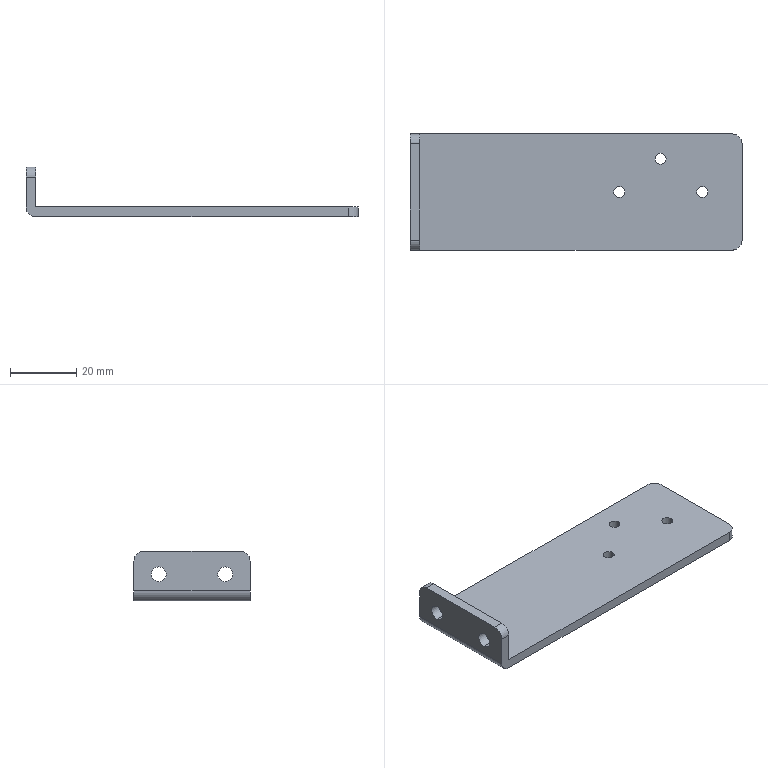Component | SolidWorks | H2020022-0443-1-1 | 1 solid | 23 faces | box 100 x 35 x 15 mm | volume 11497 mm3 | cylinder 15 | plane 8 | commonest cylinder face diameters 3.3 x6 6 x5 4.5 x4 | material Stainless Steel304
build123d program:
from build123d import *

# Parameters (mm, degrees)
BOSS_EXTRUDE1_DEPTH = 35
FILLET1_R           = 3
SKETCH2_R           = 2.25
CUT_EXTRUDE1_DEPTH  = 105.207
M4_TAPPED_HOLE1_D   = 3.3


with BuildPart() as part:
    # Sketch1 → Boss-Extrude1 (new body)
    with BuildSketch(Plane(origin=(0, 0, 0), x_dir=(1, 0, 0), z_dir=(0, 1, 0))):
        Polygon((0, 0), (0, -100), (-3, -100), (-3, -3), (-15, -3), (-15, 0), align=None)
    extrude(amount=BOSS_EXTRUDE1_DEPTH)

    # Fillet1
    fillet1_edges = [part.edges().sort_by_distance(p)[0] for p in [
        (0, 17.5, 0),
        (-1.5, 35, 100),
        (-1.5, 0, 100),
        (-15, 35, 1.5),
        (-15, 0, 1.5),
    ]]
    fillet(fillet1_edges, radius=FILLET1_R)

    # Sketch2 → Cut-Extrude1 (cut, through all)
    with BuildSketch(Plane.XY.offset(3)):
        with Locations((-8, 27.5)):
            Circle(SKETCH2_R)
        with Locations((-8, 7.5)):
            Circle(SKETCH2_R)
    extrude(amount=-CUT_EXTRUDE1_DEPTH, mode=Mode.SUBTRACT)

    # M4 Tapped Hole1 (through all)
    with Locations(Plane.ZY.offset(3)):
        with Locations((88, 17.5), (63, 17.5), (75.5, 27.5)):
            Hole(M4_TAPPED_HOLE1_D / 2)


solid = part.part

# Placed as in the assembly
solid = solid.moved(Location((11.932, 58.313, 375.197), (0, 90, 0)))
STEP:
#1=COLOUR_RGB('',0.7922,0.8196,0.9333);
#2=FILL_AREA_STYLE_COLOUR('',#1);
#3=FILL_AREA_STYLE('',(#2));
#4=SURFACE_STYLE_FILL_AREA(#3);
#5=SURFACE_SIDE_STYLE('',(#4));
#6=SURFACE_STYLE_USAGE(.BOTH.,#5);
#7=PRESENTATION_STYLE_ASSIGNMENT((#6));
#8=CARTESIAN_POINT('',(3.869,2.985,14.772));
#9=VERTEX_POINT('',#8);
#10=CARTESIAN_POINT('',(3.999,2.985,14.772));
#11=VERTEX_POINT('',#10);
#12=CARTESIAN_POINT('',(3.934,2.985,14.772));
#13=DIRECTION('',(-0.,0.,1.));
#14=DIRECTION('',(1.,0.,0.));
#15=AXIS2_PLACEMENT_3D('',#12,#13,#14);
#16=CIRCLE('',#15,0.06496);
#17=EDGE_CURVE('',#9,#11,#16,.T.);
#18=ORIENTED_EDGE('',*,*,#17,.F.);
#19=CARTESIAN_POINT('',(3.869,2.985,14.89));
#20=VERTEX_POINT('',#19);
#21=CARTESIAN_POINT('',(3.869,2.985,14.89));
#22=DIRECTION('',(-0.,0.,1.));
#23=VECTOR('',#22,39.37);
#24=LINE('',#21,#23);
#25=EDGE_CURVE('',#9,#20,#24,.T.);
#26=ORIENTED_EDGE('',*,*,#25,.T.);
#27=CARTESIAN_POINT('',(3.999,2.985,14.89));
#28=VERTEX_POINT('',#27);
#29=CARTESIAN_POINT('',(3.934,2.985,14.89));
#30=DIRECTION('',(-0.,0.,1.));
#31=DIRECTION('',(1.,0.,0.));
#32=AXIS2_PLACEMENT_3D('',#29,#30,#31);
#33=CIRCLE('',#32,0.06496);
#34=EDGE_CURVE('',#20,#28,#33,.T.);
#35=ORIENTED_EDGE('',*,*,#34,.T.);
#36=CARTESIAN_POINT('',(3.999,2.985,14.89));
#37=DIRECTION('',(-0.,0.,1.));
#38=VECTOR('',#37,39.37);
#39=LINE('',#36,#38);
#40=EDGE_CURVE('',#11,#28,#39,.T.);
#41=ORIENTED_EDGE('',*,*,#40,.F.);
#42=EDGE_LOOP('',(#18,#26,#35,#41));
#43=FACE_OUTER_BOUND('',#42,.T.);
#44=CARTESIAN_POINT('',(3.934,2.985,14.89));
#45=DIRECTION('',(-0.,0.,1.));
#46=DIRECTION('',(1.,0.,0.));
#47=AXIS2_PLACEMENT_3D('',#44,#45,#46);
#48=CYLINDRICAL_SURFACE('',#47,0.06496);
#49=ADVANCED_FACE('',(#43),#48,.F.);
#50=CARTESIAN_POINT('',(2.885,2.985,14.772));
#51=VERTEX_POINT('',#50);
#52=CARTESIAN_POINT('',(3.015,2.985,14.772));
#53=VERTEX_POINT('',#52);
#54=CARTESIAN_POINT('',(2.95,2.985,14.772));
#55=DIRECTION('',(-0.,0.,1.));
#56=DIRECTION('',(1.,0.,0.));
#57=AXIS2_PLACEMENT_3D('',#54,#55,#56);
#58=CIRCLE('',#57,0.06496);
#59=EDGE_CURVE('',#51,#53,#58,.T.);
#60=ORIENTED_EDGE('',*,*,#59,.F.);
#61=CARTESIAN_POINT('',(2.885,2.985,14.89));
#62=VERTEX_POINT('',#61);
#63=CARTESIAN_POINT('',(2.885,2.985,14.89));
#64=DIRECTION('',(-0.,0.,1.));
#65=VECTOR('',#64,39.37);
#66=LINE('',#63,#65);
#67=EDGE_CURVE('',#51,#62,#66,.T.);
#68=ORIENTED_EDGE('',*,*,#67,.T.);
#69=CARTESIAN_POINT('',(3.015,2.985,14.89));
#70=VERTEX_POINT('',#69);
#71=CARTESIAN_POINT('',(2.95,2.985,14.89));
#72=DIRECTION('',(-0.,0.,1.));
#73=DIRECTION('',(1.,0.,0.));
#74=AXIS2_PLACEMENT_3D('',#71,#72,#73);
#75=CIRCLE('',#74,0.06496);
#76=EDGE_CURVE('',#62,#70,#75,.T.);
#77=ORIENTED_EDGE('',*,*,#76,.T.);
#78=CARTESIAN_POINT('',(3.015,2.985,14.89));
#79=DIRECTION('',(-0.,0.,1.));
#80=VECTOR('',#79,39.37);
#81=LINE('',#78,#80);
#82=EDGE_CURVE('',#53,#70,#81,.T.);
#83=ORIENTED_EDGE('',*,*,#82,.F.);
#84=EDGE_LOOP('',(#60,#68,#77,#83));
#85=FACE_OUTER_BOUND('',#84,.T.);
#86=CARTESIAN_POINT('',(2.95,2.985,14.89));
#87=DIRECTION('',(-0.,0.,1.));
#88=DIRECTION('',(1.,0.,0.));
#89=AXIS2_PLACEMENT_3D('',#86,#87,#88);
#90=CYLINDRICAL_SURFACE('',#89,0.06496);
#91=ADVANCED_FACE('',(#85),#90,.F.);
#92=CARTESIAN_POINT('',(3.377,3.378,14.772));
#93=VERTEX_POINT('',#92);
#94=CARTESIAN_POINT('',(3.507,3.378,14.772));
#95=VERTEX_POINT('',#94);
#96=CARTESIAN_POINT('',(3.442,3.378,14.772));
#97=DIRECTION('',(-0.,0.,1.));
#98=DIRECTION('',(1.,0.,0.));
#99=AXIS2_PLACEMENT_3D('',#96,#97,#98);
#100=CIRCLE('',#99,0.06496);
#101=EDGE_CURVE('',#93,#95,#100,.T.);
#102=ORIENTED_EDGE('',*,*,#101,.F.);
#103=CARTESIAN_POINT('',(3.377,3.378,14.89));
#104=VERTEX_POINT('',#103);
#105=CARTESIAN_POINT('',(3.377,3.378,14.89));
#106=DIRECTION('',(-0.,0.,1.));
#107=VECTOR('',#106,39.37);
#108=LINE('',#105,#107);
#109=EDGE_CURVE('',#93,#104,#108,.T.);
#110=ORIENTED_EDGE('',*,*,#109,.T.);
#111=CARTESIAN_POINT('',(3.507,3.378,14.89));
#112=VERTEX_POINT('',#111);
#113=CARTESIAN_POINT('',(3.442,3.378,14.89));
#114=DIRECTION('',(-0.,0.,1.));
#115=DIRECTION('',(1.,0.,0.));
#116=AXIS2_PLACEMENT_3D('',#113,#114,#115);
#117=CIRCLE('',#116,0.06496);
#118=EDGE_CURVE('',#104,#112,#117,.T.);
#119=ORIENTED_EDGE('',*,*,#118,.T.);
#120=CARTESIAN_POINT('',(3.507,3.378,14.89));
#121=DIRECTION('',(-0.,0.,1.));
#122=VECTOR('',#121,39.37);
#123=LINE('',#120,#122);
#124=EDGE_CURVE('',#95,#112,#123,.T.);
#125=ORIENTED_EDGE('',*,*,#124,.F.);
#126=EDGE_LOOP('',(#102,#110,#119,#125));
#127=FACE_OUTER_BOUND('',#126,.T.);
#128=CARTESIAN_POINT('',(3.442,3.378,14.89));
#129=DIRECTION('',(-0.,0.,1.));
#130=DIRECTION('',(1.,0.,0.));
#131=AXIS2_PLACEMENT_3D('',#128,#129,#130);
#132=CYLINDRICAL_SURFACE('',#131,0.06496);
#133=ADVANCED_FACE('',(#127),#132,.F.);
#134=CARTESIAN_POINT('',(0.4697,3.378,15.175));
#135=VERTEX_POINT('',#134);
#136=CARTESIAN_POINT('',(0.4697,3.378,14.998));
#137=VERTEX_POINT('',#136);
#138=CARTESIAN_POINT('',(0.4697,3.378,15.086));
#139=DIRECTION('',(1.,0.,0.));
#140=DIRECTION('',(0.,0.,-1.));
#141=AXIS2_PLACEMENT_3D('',#138,#139,#140);
#142=CIRCLE('',#141,0.08858);
#143=EDGE_CURVE('',#135,#137,#142,.T.);
#144=ORIENTED_EDGE('',*,*,#143,.F.);
#145=CARTESIAN_POINT('',(0.5879,3.378,15.175));
#146=VERTEX_POINT('',#145);
#147=CARTESIAN_POINT('',(0.4697,3.378,15.175));
#148=DIRECTION('',(1.,0.,0.));
#149=VECTOR('',#148,39.37);
#150=LINE('',#147,#149);
#151=EDGE_CURVE('',#135,#146,#150,.T.);
#152=ORIENTED_EDGE('',*,*,#151,.T.);
#153=CARTESIAN_POINT('',(0.5879,3.378,14.998));
#154=VERTEX_POINT('',#153);
#155=CARTESIAN_POINT('',(0.5879,3.378,15.086));
#156=DIRECTION('',(1.,0.,0.));
#157=DIRECTION('',(0.,0.,-1.));
#158=AXIS2_PLACEMENT_3D('',#155,#156,#157);
#159=CIRCLE('',#158,0.08858);
#160=EDGE_CURVE('',#146,#154,#159,.T.);
#161=ORIENTED_EDGE('',*,*,#160,.T.);
#162=CARTESIAN_POINT('',(0.4697,3.378,14.998));
#163=DIRECTION('',(1.,0.,0.));
#164=VECTOR('',#163,39.37);
#165=LINE('',#162,#164);
#166=EDGE_CURVE('',#137,#154,#165,.T.);
#167=ORIENTED_EDGE('',*,*,#166,.F.);
#168=EDGE_LOOP('',(#144,#152,#161,#167));
#169=FACE_OUTER_BOUND('',#168,.T.);
#170=CARTESIAN_POINT('',(0.4697,3.378,15.086));
#171=DIRECTION('',(1.,0.,0.));
#172=DIRECTION('',(0.,0.,-1.));
#173=AXIS2_PLACEMENT_3D('',#170,#171,#172);
#174=CYLINDRICAL_SURFACE('',#173,0.08858);
#175=ADVANCED_FACE('',(#169),#174,.F.);
#176=CARTESIAN_POINT('',(0.4697,2.591,15.175));
#177=VERTEX_POINT('',#176);
#178=CARTESIAN_POINT('',(0.4697,2.591,14.998));
#179=VERTEX_POINT('',#178);
#180=CARTESIAN_POINT('',(0.4697,2.591,15.086));
#181=DIRECTION('',(1.,0.,0.));
#182=DIRECTION('',(0.,0.,-1.));
#183=AXIS2_PLACEMENT_3D('',#180,#181,#182);
#184=CIRCLE('',#183,0.08858);
#185=EDGE_CURVE('',#177,#179,#184,.T.);
#186=ORIENTED_EDGE('',*,*,#185,.F.);
#187=CARTESIAN_POINT('',(0.5879,2.591,15.175));
#188=VERTEX_POINT('',#187);
#189=CARTESIAN_POINT('',(0.4697,2.591,15.175));
#190=DIRECTION('',(1.,0.,0.));
#191=VECTOR('',#190,39.37);
#192=LINE('',#189,#191);
#193=EDGE_CURVE('',#177,#188,#192,.T.);
#194=ORIENTED_EDGE('',*,*,#193,.T.);
#195=CARTESIAN_POINT('',(0.5879,2.591,14.998));
#196=VERTEX_POINT('',#195);
#197=CARTESIAN_POINT('',(0.5879,2.591,15.086));
#198=DIRECTION('',(1.,0.,0.));
#199=DIRECTION('',(0.,0.,-1.));
#200=AXIS2_PLACEMENT_3D('',#197,#198,#199);
#201=CIRCLE('',#200,0.08858);
#202=EDGE_CURVE('',#188,#196,#201,.T.);
#203=ORIENTED_EDGE('',*,*,#202,.T.);
#204=CARTESIAN_POINT('',(0.4697,2.591,14.998));
#205=DIRECTION('',(1.,0.,0.));
#206=VECTOR('',#205,39.37);
#207=LINE('',#204,#206);
#208=EDGE_CURVE('',#179,#196,#207,.T.);
#209=ORIENTED_EDGE('',*,*,#208,.F.);
#210=EDGE_LOOP('',(#186,#194,#203,#209));
#211=FACE_OUTER_BOUND('',#210,.T.);
#212=CARTESIAN_POINT('',(0.4697,2.591,15.086));
#213=DIRECTION('',(1.,0.,0.));
#214=DIRECTION('',(0.,0.,-1.));
#215=AXIS2_PLACEMENT_3D('',#212,#213,#214);
#216=CYLINDRICAL_SURFACE('',#215,0.08858);
#217=ADVANCED_FACE('',(#211),#216,.F.);
#218=CARTESIAN_POINT('',(0.4697,3.378,15.086));
#219=DIRECTION('',(1.,0.,0.));
#220=DIRECTION('',(0.,0.,-1.));
#221=AXIS2_PLACEMENT_3D('',#218,#219,#220);
#222=CIRCLE('',#221,0.08858);
#223=EDGE_CURVE('',#137,#135,#222,.T.);
#224=ORIENTED_EDGE('',*,*,#223,.T.);
#225=ORIENTED_EDGE('',*,*,#143,.T.);
#226=EDGE_LOOP('',(#224,#225));
#227=FACE_BOUND('',#226,.T.);
#228=CARTESIAN_POINT('',(0.4697,2.591,15.086));
#229=DIRECTION('',(1.,0.,0.));
#230=DIRECTION('',(0.,0.,-1.));
#231=AXIS2_PLACEMENT_3D('',#228,#229,#230);
#232=CIRCLE('',#231,0.08858);
#233=EDGE_CURVE('',#179,#177,#232,.T.);
#234=ORIENTED_EDGE('',*,*,#233,.T.);
#235=ORIENTED_EDGE('',*,*,#185,.T.);
#236=EDGE_LOOP('',(#234,#235));
#237=FACE_BOUND('',#236,.T.);
#238=CARTESIAN_POINT('',(0.4697,2.296,14.89));
#239=VERTEX_POINT('',#238);
#240=CARTESIAN_POINT('',(0.4697,2.296,15.244));
#241=VERTEX_POINT('',#240);
#242=CARTESIAN_POINT('',(0.4697,2.296,15.362));
#243=DIRECTION('',(-0.,0.,1.));
#244=VECTOR('',#243,39.37);
#245=LINE('',#242,#244);
#246=EDGE_CURVE('',#239,#241,#245,.T.);
#247=ORIENTED_EDGE('',*,*,#246,.T.);
#248=CARTESIAN_POINT('',(0.4697,2.414,15.362));
#249=VERTEX_POINT('',#248);
#250=CARTESIAN_POINT('',(0.4697,2.414,15.244));
#251=DIRECTION('',(-1.,-0.,-0.));
#252=DIRECTION('',(0.,0.,-1.));
#253=AXIS2_PLACEMENT_3D('',#250,#251,#252);
#254=CIRCLE('',#253,0.1181);
#255=EDGE_CURVE('',#241,#249,#254,.T.);
#256=ORIENTED_EDGE('',*,*,#255,.T.);
#257=CARTESIAN_POINT('',(0.4697,3.556,15.362));
#258=VERTEX_POINT('',#257);
#259=CARTESIAN_POINT('',(0.4697,3.674,15.362));
#260=DIRECTION('',(0.,-1.,0.));
#261=VECTOR('',#260,39.37);
#262=LINE('',#259,#261);
#263=EDGE_CURVE('',#258,#249,#262,.T.);
#264=ORIENTED_EDGE('',*,*,#263,.F.);
#265=CARTESIAN_POINT('',(0.4697,3.674,15.244));
#266=VERTEX_POINT('',#265);
#267=CARTESIAN_POINT('',(0.4697,3.556,15.244));
#268=DIRECTION('',(-1.,-0.,-0.));
#269=DIRECTION('',(0.,0.,-1.));
#270=AXIS2_PLACEMENT_3D('',#267,#268,#269);
#271=CIRCLE('',#270,0.1181);
#272=EDGE_CURVE('',#258,#266,#271,.T.);
#273=ORIENTED_EDGE('',*,*,#272,.T.);
#274=CARTESIAN_POINT('',(0.4697,3.674,14.89));
#275=VERTEX_POINT('',#274);
#276=CARTESIAN_POINT('',(0.4697,3.674,15.362));
#277=DIRECTION('',(-0.,0.,1.));
#278=VECTOR('',#277,39.37);
#279=LINE('',#276,#278);
#280=EDGE_CURVE('',#275,#266,#279,.T.);
#281=ORIENTED_EDGE('',*,*,#280,.F.);
#282=CARTESIAN_POINT('',(0.4697,3.674,14.89));
#283=DIRECTION('',(0.,-1.,0.));
#284=VECTOR('',#283,39.37);
#285=LINE('',#282,#284);
#286=EDGE_CURVE('',#275,#239,#285,.T.);
#287=ORIENTED_EDGE('',*,*,#286,.T.);
#288=EDGE_LOOP('',(#247,#256,#264,#273,#281,#287));
#289=FACE_OUTER_BOUND('',#288,.T.);
#290=CARTESIAN_POINT('',(0.4697,3.674,15.362));
#291=DIRECTION('',(1.,0.,0.));
#292=DIRECTION('',(0.,-0.,-1.));
#293=AXIS2_PLACEMENT_3D('',#290,#291,#292);
#294=PLANE('',#293);
#295=ADVANCED_FACE('',(#227,#237,#289),#294,.F.);
#296=ORIENTED_EDGE('',*,*,#263,.T.);
#297=CARTESIAN_POINT('',(0.5879,2.414,15.362));
#298=VERTEX_POINT('',#297);
#299=CARTESIAN_POINT('',(0.5879,2.414,15.362));
#300=DIRECTION('',(1.,0.,0.));
#301=VECTOR('',#300,39.37);
#302=LINE('',#299,#301);
#303=EDGE_CURVE('',#249,#298,#302,.T.);
#304=ORIENTED_EDGE('',*,*,#303,.T.);
#305=CARTESIAN_POINT('',(0.5879,3.556,15.362));
#306=VERTEX_POINT('',#305);
#307=CARTESIAN_POINT('',(0.5879,3.674,15.362));
#308=DIRECTION('',(0.,-1.,0.));
#309=VECTOR('',#308,39.37);
#310=LINE('',#307,#309);
#311=EDGE_CURVE('',#306,#298,#310,.T.);
#312=ORIENTED_EDGE('',*,*,#311,.F.);
#313=CARTESIAN_POINT('',(0.5879,3.556,15.362));
#314=DIRECTION('',(-1.,-0.,-0.));
#315=VECTOR('',#314,39.37);
#316=LINE('',#313,#315);
#317=EDGE_CURVE('',#306,#258,#316,.T.);
#318=ORIENTED_EDGE('',*,*,#317,.T.);
#319=EDGE_LOOP('',(#296,#304,#312,#318));
#320=FACE_OUTER_BOUND('',#319,.T.);
#321=CARTESIAN_POINT('',(0.5879,3.674,15.362));
#322=DIRECTION('',(0.,-0.,-1.));
#323=DIRECTION('',(-1.,-0.,-0.));
#324=AXIS2_PLACEMENT_3D('',#321,#322,#323);
#325=PLANE('',#324);
#326=ADVANCED_FACE('',(#320),#325,.F.);
#327=CARTESIAN_POINT('',(0.5879,3.378,15.086));
#328=DIRECTION('',(1.,0.,0.));
#329=DIRECTION('',(0.,0.,-1.));
#330=AXIS2_PLACEMENT_3D('',#327,#328,#329);
#331=CIRCLE('',#330,0.08858);
#332=EDGE_CURVE('',#154,#146,#331,.T.);
#333=ORIENTED_EDGE('',*,*,#332,.F.);
#334=ORIENTED_EDGE('',*,*,#160,.F.);
#335=EDGE_LOOP('',(#333,#334));
#336=FACE_BOUND('',#335,.T.);
#337=CARTESIAN_POINT('',(0.5879,2.591,15.086));
#338=DIRECTION('',(1.,0.,0.));
#339=DIRECTION('',(0.,0.,-1.));
#340=AXIS2_PLACEMENT_3D('',#337,#338,#339);
#341=CIRCLE('',#340,0.08858);
#342=EDGE_CURVE('',#196,#188,#341,.T.);
#343=ORIENTED_EDGE('',*,*,#342,.F.);
#344=ORIENTED_EDGE('',*,*,#202,.F.);
#345=EDGE_LOOP('',(#343,#344));
#346=FACE_BOUND('',#345,.T.);
#347=ORIENTED_EDGE('',*,*,#311,.T.);
#348=CARTESIAN_POINT('',(0.5879,2.296,15.244));
#349=VERTEX_POINT('',#348);
#350=CARTESIAN_POINT('',(0.5879,2.414,15.244));
#351=DIRECTION('',(1.,0.,-0.));
#352=DIRECTION('',(0.,0.,1.));
#353=AXIS2_PLACEMENT_3D('',#350,#351,#352);
#354=CIRCLE('',#353,0.1181);
#355=EDGE_CURVE('',#298,#349,#354,.T.);
#356=ORIENTED_EDGE('',*,*,#355,.T.);
#357=CARTESIAN_POINT('',(0.5879,2.296,14.89));
#358=VERTEX_POINT('',#357);
#359=CARTESIAN_POINT('',(0.5879,2.296,14.89));
#360=DIRECTION('',(-0.,-0.,-1.));
#361=VECTOR('',#360,39.37);
#362=LINE('',#359,#361);
#363=EDGE_CURVE('',#349,#358,#362,.T.);
#364=ORIENTED_EDGE('',*,*,#363,.T.);
#365=CARTESIAN_POINT('',(0.5879,3.674,14.89));
#366=VERTEX_POINT('',#365);
#367=CARTESIAN_POINT('',(0.5879,3.674,14.89));
#368=DIRECTION('',(0.,-1.,0.));
#369=VECTOR('',#368,39.37);
#370=LINE('',#367,#369);
#371=EDGE_CURVE('',#366,#358,#370,.T.);
#372=ORIENTED_EDGE('',*,*,#371,.F.);
#373=CARTESIAN_POINT('',(0.5879,3.674,15.244));
#374=VERTEX_POINT('',#373);
#375=CARTESIAN_POINT('',(0.5879,3.674,14.89));
#376=DIRECTION('',(-0.,-0.,-1.));
#377=VECTOR('',#376,39.37);
#378=LINE('',#375,#377);
#379=EDGE_CURVE('',#374,#366,#378,.T.);
#380=ORIENTED_EDGE('',*,*,#379,.F.);
#381=CARTESIAN_POINT('',(0.5879,3.556,15.244));
#382=DIRECTION('',(1.,0.,-0.));
#383=DIRECTION('',(0.,0.,1.));
#384=AXIS2_PLACEMENT_3D('',#381,#382,#383);
#385=CIRCLE('',#384,0.1181);
#386=EDGE_CURVE('',#374,#306,#385,.T.);
#387=ORIENTED_EDGE('',*,*,#386,.T.);
#388=EDGE_LOOP('',(#347,#356,#364,#372,#380,#387));
#389=FACE_OUTER_BOUND('',#388,.T.);
#390=CARTESIAN_POINT('',(0.5879,3.674,14.89));
#391=DIRECTION('',(-1.,-0.,0.));
#392=DIRECTION('',(0.,0.,1.));
#393=AXIS2_PLACEMENT_3D('',#390,#391,#392);
#394=PLANE('',#393);
#395=ADVANCED_FACE('',(#336,#346,#389),#394,.F.);
#396=CARTESIAN_POINT('',(3.934,2.985,14.89));
#397=DIRECTION('',(-0.,0.,1.));
#398=DIRECTION('',(1.,0.,0.));
#399=AXIS2_PLACEMENT_3D('',#396,#397,#398);
#400=CIRCLE('',#399,0.06496);
#401=EDGE_CURVE('',#28,#20,#400,.T.);
#402=ORIENTED_EDGE('',*,*,#401,.F.);
#403=ORIENTED_EDGE('',*,*,#34,.F.);
#404=EDGE_LOOP('',(#402,#403));
#405=FACE_BOUND('',#404,.T.);
#406=CARTESIAN_POINT('',(2.95,2.985,14.89));
#407=DIRECTION('',(-0.,0.,1.));
#408=DIRECTION('',(1.,0.,0.));
#409=AXIS2_PLACEMENT_3D('',#406,#407,#408);
#410=CIRCLE('',#409,0.06496);
#411=EDGE_CURVE('',#70,#62,#410,.T.);
#412=ORIENTED_EDGE('',*,*,#411,.F.);
#413=ORIENTED_EDGE('',*,*,#76,.F.);
#414=EDGE_LOOP('',(#412,#413));
#415=FACE_BOUND('',#414,.T.);
#416=CARTESIAN_POINT('',(3.442,3.378,14.89));
#417=DIRECTION('',(-0.,0.,1.));
#418=DIRECTION('',(1.,0.,0.));
#419=AXIS2_PLACEMENT_3D('',#416,#417,#418);
#420=CIRCLE('',#419,0.06496);
#421=EDGE_CURVE('',#112,#104,#420,.T.);
#422=ORIENTED_EDGE('',*,*,#421,.F.);
#423=ORIENTED_EDGE('',*,*,#118,.F.);
#424=EDGE_LOOP('',(#422,#423));
#425=FACE_BOUND('',#424,.T.);
#426=CARTESIAN_POINT('',(4.407,3.556,14.89));
#427=VERTEX_POINT('',#426);
#428=CARTESIAN_POINT('',(4.407,2.414,14.89));
#429=VERTEX_POINT('',#428);
#430=CARTESIAN_POINT('',(4.407,3.674,14.89));
#431=DIRECTION('',(0.,-1.,0.));
#432=VECTOR('',#431,39.37);
#433=LINE('',#430,#432);
#434=EDGE_CURVE('',#427,#429,#433,.T.);
#435=ORIENTED_EDGE('',*,*,#434,.F.);
#436=CARTESIAN_POINT('',(4.289,3.674,14.89));
#437=VERTEX_POINT('',#436);
#438=CARTESIAN_POINT('',(4.289,3.556,14.89));
#439=DIRECTION('',(-0.,0.,1.));
#440=DIRECTION('',(-1.,0.,0.));
#441=AXIS2_PLACEMENT_3D('',#438,#439,#440);
#442=CIRCLE('',#441,0.1181);
#443=EDGE_CURVE('',#427,#437,#442,.T.);
#444=ORIENTED_EDGE('',*,*,#443,.T.);
#445=CARTESIAN_POINT('',(4.407,3.674,14.89));
#446=DIRECTION('',(1.,0.,0.));
#447=VECTOR('',#446,39.37);
#448=LINE('',#445,#447);
#449=EDGE_CURVE('',#366,#437,#448,.T.);
#450=ORIENTED_EDGE('',*,*,#449,.F.);
#451=ORIENTED_EDGE('',*,*,#371,.T.);
#452=CARTESIAN_POINT('',(4.289,2.296,14.89));
#453=VERTEX_POINT('',#452);
#454=CARTESIAN_POINT('',(4.407,2.296,14.89));
#455=DIRECTION('',(1.,0.,0.));
#456=VECTOR('',#455,39.37);
#457=LINE('',#454,#456);
#458=EDGE_CURVE('',#358,#453,#457,.T.);
#459=ORIENTED_EDGE('',*,*,#458,.T.);
#460=CARTESIAN_POINT('',(4.289,2.414,14.89));
#461=DIRECTION('',(-0.,0.,1.));
#462=DIRECTION('',(-1.,0.,0.));
#463=AXIS2_PLACEMENT_3D('',#460,#461,#462);
#464=CIRCLE('',#463,0.1181);
#465=EDGE_CURVE('',#453,#429,#464,.T.);
#466=ORIENTED_EDGE('',*,*,#465,.T.);
#467=EDGE_LOOP('',(#435,#444,#450,#451,#459,#466));
#468=FACE_OUTER_BOUND('',#467,.T.);
#469=CARTESIAN_POINT('',(4.407,3.674,14.89));
#470=DIRECTION('',(0.,-0.,-1.));
#471=DIRECTION('',(-1.,-0.,-0.));
#472=AXIS2_PLACEMENT_3D('',#469,#470,#471);
#473=PLANE('',#472);
#474=ADVANCED_FACE('',(#405,#415,#425,#468),#473,.F.);
#475=CARTESIAN_POINT('',(4.407,3.556,14.772));
#476=VERTEX_POINT('',#475);
#477=CARTESIAN_POINT('',(4.407,2.414,14.772));
#478=VERTEX_POINT('',#477);
#479=CARTESIAN_POINT('',(4.407,3.674,14.772));
#480=DIRECTION('',(0.,-1.,0.));
#481=VECTOR('',#480,39.37);
#482=LINE('',#479,#481);
#483=EDGE_CURVE('',#476,#478,#482,.T.);
#484=ORIENTED_EDGE('',*,*,#483,.F.);
#485=CARTESIAN_POINT('',(4.407,3.556,14.772));
#486=DIRECTION('',(-0.,0.,1.));
#487=VECTOR('',#486,39.37);
#488=LINE('',#485,#487);
#489=EDGE_CURVE('',#476,#427,#488,.T.);
#490=ORIENTED_EDGE('',*,*,#489,.T.);
#491=ORIENTED_EDGE('',*,*,#434,.T.);
#492=CARTESIAN_POINT('',(4.407,2.414,14.772));
#493=DIRECTION('',(0.,-0.,-1.));
#494=VECTOR('',#493,39.37);
#495=LINE('',#492,#494);
#496=EDGE_CURVE('',#429,#478,#495,.T.);
#497=ORIENTED_EDGE('',*,*,#496,.T.);
#498=EDGE_LOOP('',(#484,#490,#491,#497));
#499=FACE_OUTER_BOUND('',#498,.T.);
#500=CARTESIAN_POINT('',(4.407,3.674,14.772));
#501=DIRECTION('',(-1.,-0.,-0.));
#502=DIRECTION('',(-0.,0.,1.));
#503=AXIS2_PLACEMENT_3D('',#500,#501,#502);
#504=PLANE('',#503);
#505=ADVANCED_FACE('',(#499),#504,.F.);
#506=CARTESIAN_POINT('',(3.934,2.985,14.772));
#507=DIRECTION('',(-0.,0.,1.));
#508=DIRECTION('',(1.,0.,0.));
#509=AXIS2_PLACEMENT_3D('',#506,#507,#508);
#510=CIRCLE('',#509,0.06496);
#511=EDGE_CURVE('',#11,#9,#510,.T.);
#512=ORIENTED_EDGE('',*,*,#511,.T.);
#513=ORIENTED_EDGE('',*,*,#17,.T.);
#514=EDGE_LOOP('',(#512,#513));
#515=FACE_BOUND('',#514,.T.);
#516=CARTESIAN_POINT('',(2.95,2.985,14.772));
#517=DIRECTION('',(-0.,0.,1.));
#518=DIRECTION('',(1.,0.,0.));
#519=AXIS2_PLACEMENT_3D('',#516,#517,#518);
#520=CIRCLE('',#519,0.06496);
#521=EDGE_CURVE('',#53,#51,#520,.T.);
#522=ORIENTED_EDGE('',*,*,#521,.T.);
#523=ORIENTED_EDGE('',*,*,#59,.T.);
#524=EDGE_LOOP('',(#522,#523));
#525=FACE_BOUND('',#524,.T.);
#526=CARTESIAN_POINT('',(3.442,3.378,14.772));
#527=DIRECTION('',(-0.,0.,1.));
#528=DIRECTION('',(1.,0.,0.));
#529=AXIS2_PLACEMENT_3D('',#526,#527,#528);
#530=CIRCLE('',#529,0.06496);
#531=EDGE_CURVE('',#95,#93,#530,.T.);
#532=ORIENTED_EDGE('',*,*,#531,.T.);
#533=ORIENTED_EDGE('',*,*,#101,.T.);
#534=EDGE_LOOP('',(#532,#533));
#535=FACE_BOUND('',#534,.T.);
#536=CARTESIAN_POINT('',(4.289,3.674,14.772));
#537=VERTEX_POINT('',#536);
#538=CARTESIAN_POINT('',(0.5879,3.674,14.772));
#539=VERTEX_POINT('',#538);
#540=CARTESIAN_POINT('',(0.4697,3.674,14.772));
#541=DIRECTION('',(-1.,-0.,0.));
#542=VECTOR('',#541,39.37);
#543=LINE('',#540,#542);
#544=EDGE_CURVE('',#537,#539,#543,.T.);
#545=ORIENTED_EDGE('',*,*,#544,.F.);
#546=CARTESIAN_POINT('',(4.289,3.556,14.772));
#547=DIRECTION('',(-0.,-0.,-1.));
#548=DIRECTION('',(1.,0.,0.));
#549=AXIS2_PLACEMENT_3D('',#546,#547,#548);
#550=CIRCLE('',#549,0.1181);
#551=EDGE_CURVE('',#537,#476,#550,.T.);
#552=ORIENTED_EDGE('',*,*,#551,.T.);
#553=ORIENTED_EDGE('',*,*,#483,.T.);
#554=CARTESIAN_POINT('',(4.289,2.296,14.772));
#555=VERTEX_POINT('',#554);
#556=CARTESIAN_POINT('',(4.289,2.414,14.772));
#557=DIRECTION('',(-0.,-0.,-1.));
#558=DIRECTION('',(1.,0.,0.));
#559=AXIS2_PLACEMENT_3D('',#556,#557,#558);
#560=CIRCLE('',#559,0.1181);
#561=EDGE_CURVE('',#478,#555,#560,.T.);
#562=ORIENTED_EDGE('',*,*,#561,.T.);
#563=CARTESIAN_POINT('',(0.5879,2.296,14.772));
#564=VERTEX_POINT('',#563);
#565=CARTESIAN_POINT('',(0.4697,2.296,14.772));
#566=DIRECTION('',(-1.,-0.,0.));
#567=VECTOR('',#566,39.37);
#568=LINE('',#565,#567);
#569=EDGE_CURVE('',#555,#564,#568,.T.);
#570=ORIENTED_EDGE('',*,*,#569,.T.);
#571=CARTESIAN_POINT('',(0.5879,3.674,14.772));
#572=DIRECTION('',(-0.,1.,-0.));
#573=VECTOR('',#572,39.37);
#574=LINE('',#571,#573);
#575=EDGE_CURVE('',#564,#539,#574,.T.);
#576=ORIENTED_EDGE('',*,*,#575,.T.);
#577=EDGE_LOOP('',(#545,#552,#553,#562,#570,#576));
#578=FACE_OUTER_BOUND('',#577,.T.);
#579=CARTESIAN_POINT('',(0.4697,3.674,14.772));
#580=DIRECTION('',(0.,0.,1.));
#581=DIRECTION('',(1.,0.,-0.));
#582=AXIS2_PLACEMENT_3D('',#579,#580,#581);
#583=PLANE('',#582);
#584=ADVANCED_FACE('',(#515,#525,#535,#578),#583,.F.);
#585=ORIENTED_EDGE('',*,*,#449,.T.);
#586=CARTESIAN_POINT('',(4.289,3.674,14.772));
#587=DIRECTION('',(0.,-0.,-1.));
#588=VECTOR('',#587,39.37);
#589=LINE('',#586,#588);
#590=EDGE_CURVE('',#437,#537,#589,.T.);
#591=ORIENTED_EDGE('',*,*,#590,.T.);
#592=ORIENTED_EDGE('',*,*,#544,.T.);
#593=CARTESIAN_POINT('',(0.5879,3.674,14.89));
#594=DIRECTION('',(-0.,1.,-0.));
#595=DIRECTION('',(-1.,0.,0.));
#596=AXIS2_PLACEMENT_3D('',#593,#594,#595);
#597=CIRCLE('',#596,0.1181);
#598=EDGE_CURVE('',#539,#275,#597,.T.);
#599=ORIENTED_EDGE('',*,*,#598,.T.);
#600=ORIENTED_EDGE('',*,*,#280,.T.);
#601=CARTESIAN_POINT('',(0.4697,3.674,15.244));
#602=DIRECTION('',(1.,0.,0.));
#603=VECTOR('',#602,39.37);
#604=LINE('',#601,#603);
#605=EDGE_CURVE('',#266,#374,#604,.T.);
#606=ORIENTED_EDGE('',*,*,#605,.T.);
#607=ORIENTED_EDGE('',*,*,#379,.T.);
#608=EDGE_LOOP('',(#585,#591,#592,#599,#600,#606,#607));
#609=FACE_OUTER_BOUND('',#608,.T.);
#610=CARTESIAN_POINT('',(0.4697,3.674,14.772));
#611=DIRECTION('',(0.,-1.,0.));
#612=DIRECTION('',(-1.,-0.,-0.));
#613=AXIS2_PLACEMENT_3D('',#610,#611,#612);
#614=PLANE('',#613);
#615=ADVANCED_FACE('',(#609),#614,.F.);
#616=ORIENTED_EDGE('',*,*,#569,.F.);
#617=CARTESIAN_POINT('',(4.289,2.296,14.89));
#618=DIRECTION('',(-0.,0.,1.));
#619=VECTOR('',#618,39.37);
#620=LINE('',#617,#619);
#621=EDGE_CURVE('',#555,#453,#620,.T.);
#622=ORIENTED_EDGE('',*,*,#621,.T.);
#623=ORIENTED_EDGE('',*,*,#458,.F.);
#624=ORIENTED_EDGE('',*,*,#363,.F.);
#625=CARTESIAN_POINT('',(0.4697,2.296,15.244));
#626=DIRECTION('',(-1.,-0.,-0.));
#627=VECTOR('',#626,39.37);
#628=LINE('',#625,#627);
#629=EDGE_CURVE('',#349,#241,#628,.T.);
#630=ORIENTED_EDGE('',*,*,#629,.T.);
#631=ORIENTED_EDGE('',*,*,#246,.F.);
#632=CARTESIAN_POINT('',(0.5879,2.296,14.89));
#633=DIRECTION('',(0.,-1.,0.));
#634=DIRECTION('',(-1.,0.,0.));
#635=AXIS2_PLACEMENT_3D('',#632,#633,#634);
#636=CIRCLE('',#635,0.1181);
#637=EDGE_CURVE('',#239,#564,#636,.T.);
#638=ORIENTED_EDGE('',*,*,#637,.T.);
#639=EDGE_LOOP('',(#616,#622,#623,#624,#630,#631,#638));
#640=FACE_OUTER_BOUND('',#639,.T.);
#641=CARTESIAN_POINT('',(0.4697,2.296,14.772));
#642=DIRECTION('',(0.,-1.,0.));
#643=DIRECTION('',(-1.,-0.,-0.));
#644=AXIS2_PLACEMENT_3D('',#641,#642,#643);
#645=PLANE('',#644);
#646=ADVANCED_FACE('',(#640),#645,.T.);
#647=ORIENTED_EDGE('',*,*,#443,.F.);
#648=ORIENTED_EDGE('',*,*,#489,.F.);
#649=ORIENTED_EDGE('',*,*,#551,.F.);
#650=ORIENTED_EDGE('',*,*,#590,.F.);
#651=EDGE_LOOP('',(#647,#648,#649,#650));
#652=FACE_OUTER_BOUND('',#651,.T.);
#653=CARTESIAN_POINT('',(4.289,3.556,14.772));
#654=DIRECTION('',(0.,-0.,-1.));
#655=DIRECTION('',(-1.,0.,0.));
#656=AXIS2_PLACEMENT_3D('',#653,#654,#655);
#657=CYLINDRICAL_SURFACE('',#656,0.1181);
#658=ADVANCED_FACE('',(#652),#657,.T.);
#659=ORIENTED_EDGE('',*,*,#465,.F.);
#660=ORIENTED_EDGE('',*,*,#621,.F.);
#661=ORIENTED_EDGE('',*,*,#561,.F.);
#662=ORIENTED_EDGE('',*,*,#496,.F.);
#663=EDGE_LOOP('',(#659,#660,#661,#662));
#664=FACE_OUTER_BOUND('',#663,.T.);
#665=CARTESIAN_POINT('',(4.289,2.414,14.772));
#666=DIRECTION('',(-0.,0.,1.));
#667=DIRECTION('',(1.,0.,0.));
#668=AXIS2_PLACEMENT_3D('',#665,#666,#667);
#669=CYLINDRICAL_SURFACE('',#668,0.1181);
#670=ADVANCED_FACE('',(#664),#669,.T.);
#671=ORIENTED_EDGE('',*,*,#255,.F.);
#672=ORIENTED_EDGE('',*,*,#629,.F.);
#673=ORIENTED_EDGE('',*,*,#355,.F.);
#674=ORIENTED_EDGE('',*,*,#303,.F.);
#675=EDGE_LOOP('',(#671,#672,#673,#674));
#676=FACE_OUTER_BOUND('',#675,.T.);
#677=CARTESIAN_POINT('',(0.5879,2.414,15.244));
#678=DIRECTION('',(-1.,-0.,-0.));
#679=DIRECTION('',(0.,0.,1.));
#680=AXIS2_PLACEMENT_3D('',#677,#678,#679);
#681=CYLINDRICAL_SURFACE('',#680,0.1181);
#682=ADVANCED_FACE('',(#676),#681,.T.);
#683=ORIENTED_EDGE('',*,*,#272,.F.);
#684=ORIENTED_EDGE('',*,*,#317,.F.);
#685=ORIENTED_EDGE('',*,*,#386,.F.);
#686=ORIENTED_EDGE('',*,*,#605,.F.);
#687=EDGE_LOOP('',(#683,#684,#685,#686));
#688=FACE_OUTER_BOUND('',#687,.T.);
#689=CARTESIAN_POINT('',(0.4697,3.556,15.244));
#690=DIRECTION('',(1.,0.,0.));
#691=DIRECTION('',(0.,0.,-1.));
#692=AXIS2_PLACEMENT_3D('',#689,#690,#691);
#693=CYLINDRICAL_SURFACE('',#692,0.1181);
#694=ADVANCED_FACE('',(#688),#693,.T.);
#695=ORIENTED_EDGE('',*,*,#598,.F.);
#696=ORIENTED_EDGE('',*,*,#575,.F.);
#697=ORIENTED_EDGE('',*,*,#637,.F.);
#698=ORIENTED_EDGE('',*,*,#286,.F.);
#699=EDGE_LOOP('',(#695,#696,#697,#698));
#700=FACE_OUTER_BOUND('',#699,.T.);
#701=CARTESIAN_POINT('',(0.5879,3.674,14.89));
#702=DIRECTION('',(0.,-1.,0.));
#703=DIRECTION('',(-1.,0.,0.));
#704=AXIS2_PLACEMENT_3D('',#701,#702,#703);
#705=CYLINDRICAL_SURFACE('',#704,0.1181);
#706=ADVANCED_FACE('',(#700),#705,.T.);
#707=ORIENTED_EDGE('',*,*,#193,.F.);
#708=ORIENTED_EDGE('',*,*,#233,.F.);
#709=ORIENTED_EDGE('',*,*,#208,.T.);
#710=ORIENTED_EDGE('',*,*,#342,.T.);
#711=EDGE_LOOP('',(#707,#708,#709,#710));
#712=FACE_OUTER_BOUND('',#711,.T.);
#713=CARTESIAN_POINT('',(0.4697,2.591,15.086));
#714=DIRECTION('',(1.,0.,0.));
#715=DIRECTION('',(0.,0.,-1.));
#716=AXIS2_PLACEMENT_3D('',#713,#714,#715);
#717=CYLINDRICAL_SURFACE('',#716,0.08858);
#718=ADVANCED_FACE('',(#712),#717,.F.);
#719=ORIENTED_EDGE('',*,*,#151,.F.);
#720=ORIENTED_EDGE('',*,*,#223,.F.);
#721=ORIENTED_EDGE('',*,*,#166,.T.);
#722=ORIENTED_EDGE('',*,*,#332,.T.);
#723=EDGE_LOOP('',(#719,#720,#721,#722));
#724=FACE_OUTER_BOUND('',#723,.T.);
#725=CARTESIAN_POINT('',(0.4697,3.378,15.086));
#726=DIRECTION('',(1.,0.,0.));
#727=DIRECTION('',(0.,0.,-1.));
#728=AXIS2_PLACEMENT_3D('',#725,#726,#727);
#729=CYLINDRICAL_SURFACE('',#728,0.08858);
#730=ADVANCED_FACE('',(#724),#729,.F.);
#731=ORIENTED_EDGE('',*,*,#109,.F.);
#732=ORIENTED_EDGE('',*,*,#531,.F.);
#733=ORIENTED_EDGE('',*,*,#124,.T.);
#734=ORIENTED_EDGE('',*,*,#421,.T.);
#735=EDGE_LOOP('',(#731,#732,#733,#734));
#736=FACE_OUTER_BOUND('',#735,.T.);
#737=CARTESIAN_POINT('',(3.442,3.378,14.89));
#738=DIRECTION('',(-0.,0.,1.));
#739=DIRECTION('',(1.,0.,0.));
#740=AXIS2_PLACEMENT_3D('',#737,#738,#739);
#741=CYLINDRICAL_SURFACE('',#740,0.06496);
#742=ADVANCED_FACE('',(#736),#741,.F.);
#743=ORIENTED_EDGE('',*,*,#67,.F.);
#744=ORIENTED_EDGE('',*,*,#521,.F.);
#745=ORIENTED_EDGE('',*,*,#82,.T.);
#746=ORIENTED_EDGE('',*,*,#411,.T.);
#747=EDGE_LOOP('',(#743,#744,#745,#746));
#748=FACE_OUTER_BOUND('',#747,.T.);
#749=CARTESIAN_POINT('',(2.95,2.985,14.89));
#750=DIRECTION('',(-0.,0.,1.));
#751=DIRECTION('',(1.,0.,0.));
#752=AXIS2_PLACEMENT_3D('',#749,#750,#751);
#753=CYLINDRICAL_SURFACE('',#752,0.06496);
#754=ADVANCED_FACE('',(#748),#753,.F.);
#755=ORIENTED_EDGE('',*,*,#25,.F.);
#756=ORIENTED_EDGE('',*,*,#511,.F.);
#757=ORIENTED_EDGE('',*,*,#40,.T.);
#758=ORIENTED_EDGE('',*,*,#401,.T.);
#759=EDGE_LOOP('',(#755,#756,#757,#758));
#760=FACE_OUTER_BOUND('',#759,.T.);
#761=CARTESIAN_POINT('',(3.934,2.985,14.89));
#762=DIRECTION('',(-0.,0.,1.));
#763=DIRECTION('',(1.,0.,0.));
#764=AXIS2_PLACEMENT_3D('',#761,#762,#763);
#765=CYLINDRICAL_SURFACE('',#764,0.06496);
#766=ADVANCED_FACE('',(#760),#765,.F.);
#767=CLOSED_SHELL('',(#49,#91,#133,#175,#217,#295,#326,#395,#474,#505,#584,#615,#646,#658,#670,#682,#694,#706,#718,#730,#742,#754,#766));
#768=MANIFOLD_SOLID_BREP('',#767);
#769=STYLED_ITEM('',(#7),#768);
#770=PRESENTATION_LAYER_ASSIGNMENT('','',(#769));
#771=CARTESIAN_POINT('',(0.,0.,0.));
#772=DIRECTION('',(0.,0.,1.));
#773=DIRECTION('',(1.,0.,0.));
#774=AXIS2_PLACEMENT_3D('',#771,#772,#773);
#775=(LENGTH_UNIT()NAMED_UNIT(*)SI_UNIT($,.METRE.));
#776=LENGTH_MEASURE_WITH_UNIT(LENGTH_MEASURE(0.0254),#775);
#777=DIMENSIONAL_EXPONENTS(1.,0.,0.,0.,0.,0.,0.);
#778=(CONVERSION_BASED_UNIT('',#776)LENGTH_UNIT()NAMED_UNIT(#777));
#779=UNCERTAINTY_MEASURE_WITH_UNIT(LENGTH_MEASURE(0.00001),#778,'','');
#780=(NAMED_UNIT(*)PLANE_ANGLE_UNIT()SI_UNIT($,.RADIAN.));
#781=(NAMED_UNIT(*)SI_UNIT($,.STERADIAN.)SOLID_ANGLE_UNIT());
#782=(GEOMETRIC_REPRESENTATION_CONTEXT(3)GLOBAL_UNCERTAINTY_ASSIGNED_CONTEXT((#779))GLOBAL_UNIT_ASSIGNED_CONTEXT((#778,#780,#781))REPRESENTATION_CONTEXT('',''));
#783=ADVANCED_BREP_SHAPE_REPRESENTATION('',(#768,#774),#782);
#784=(LENGTH_UNIT()NAMED_UNIT(*)SI_UNIT($,.METRE.));
#785=LENGTH_MEASURE_WITH_UNIT(LENGTH_MEASURE(0.0254),#784);
#786=DIMENSIONAL_EXPONENTS(1.,0.,0.,0.,0.,0.,0.);
#787=(CONVERSION_BASED_UNIT('',#785)LENGTH_UNIT()NAMED_UNIT(#786));
#788=UNCERTAINTY_MEASURE_WITH_UNIT(LENGTH_MEASURE(0.00001),#787,'','');
#789=(NAMED_UNIT(*)PLANE_ANGLE_UNIT()SI_UNIT($,.RADIAN.));
#790=(NAMED_UNIT(*)SI_UNIT($,.STERADIAN.)SOLID_ANGLE_UNIT());
#791=(GEOMETRIC_REPRESENTATION_CONTEXT(3)GLOBAL_UNCERTAINTY_ASSIGNED_CONTEXT((#788))GLOBAL_UNIT_ASSIGNED_CONTEXT((#787,#789,#790))REPRESENTATION_CONTEXT('',''));
#792=MECHANICAL_DESIGN_GEOMETRIC_PRESENTATION_REPRESENTATION('',(#769),#791);